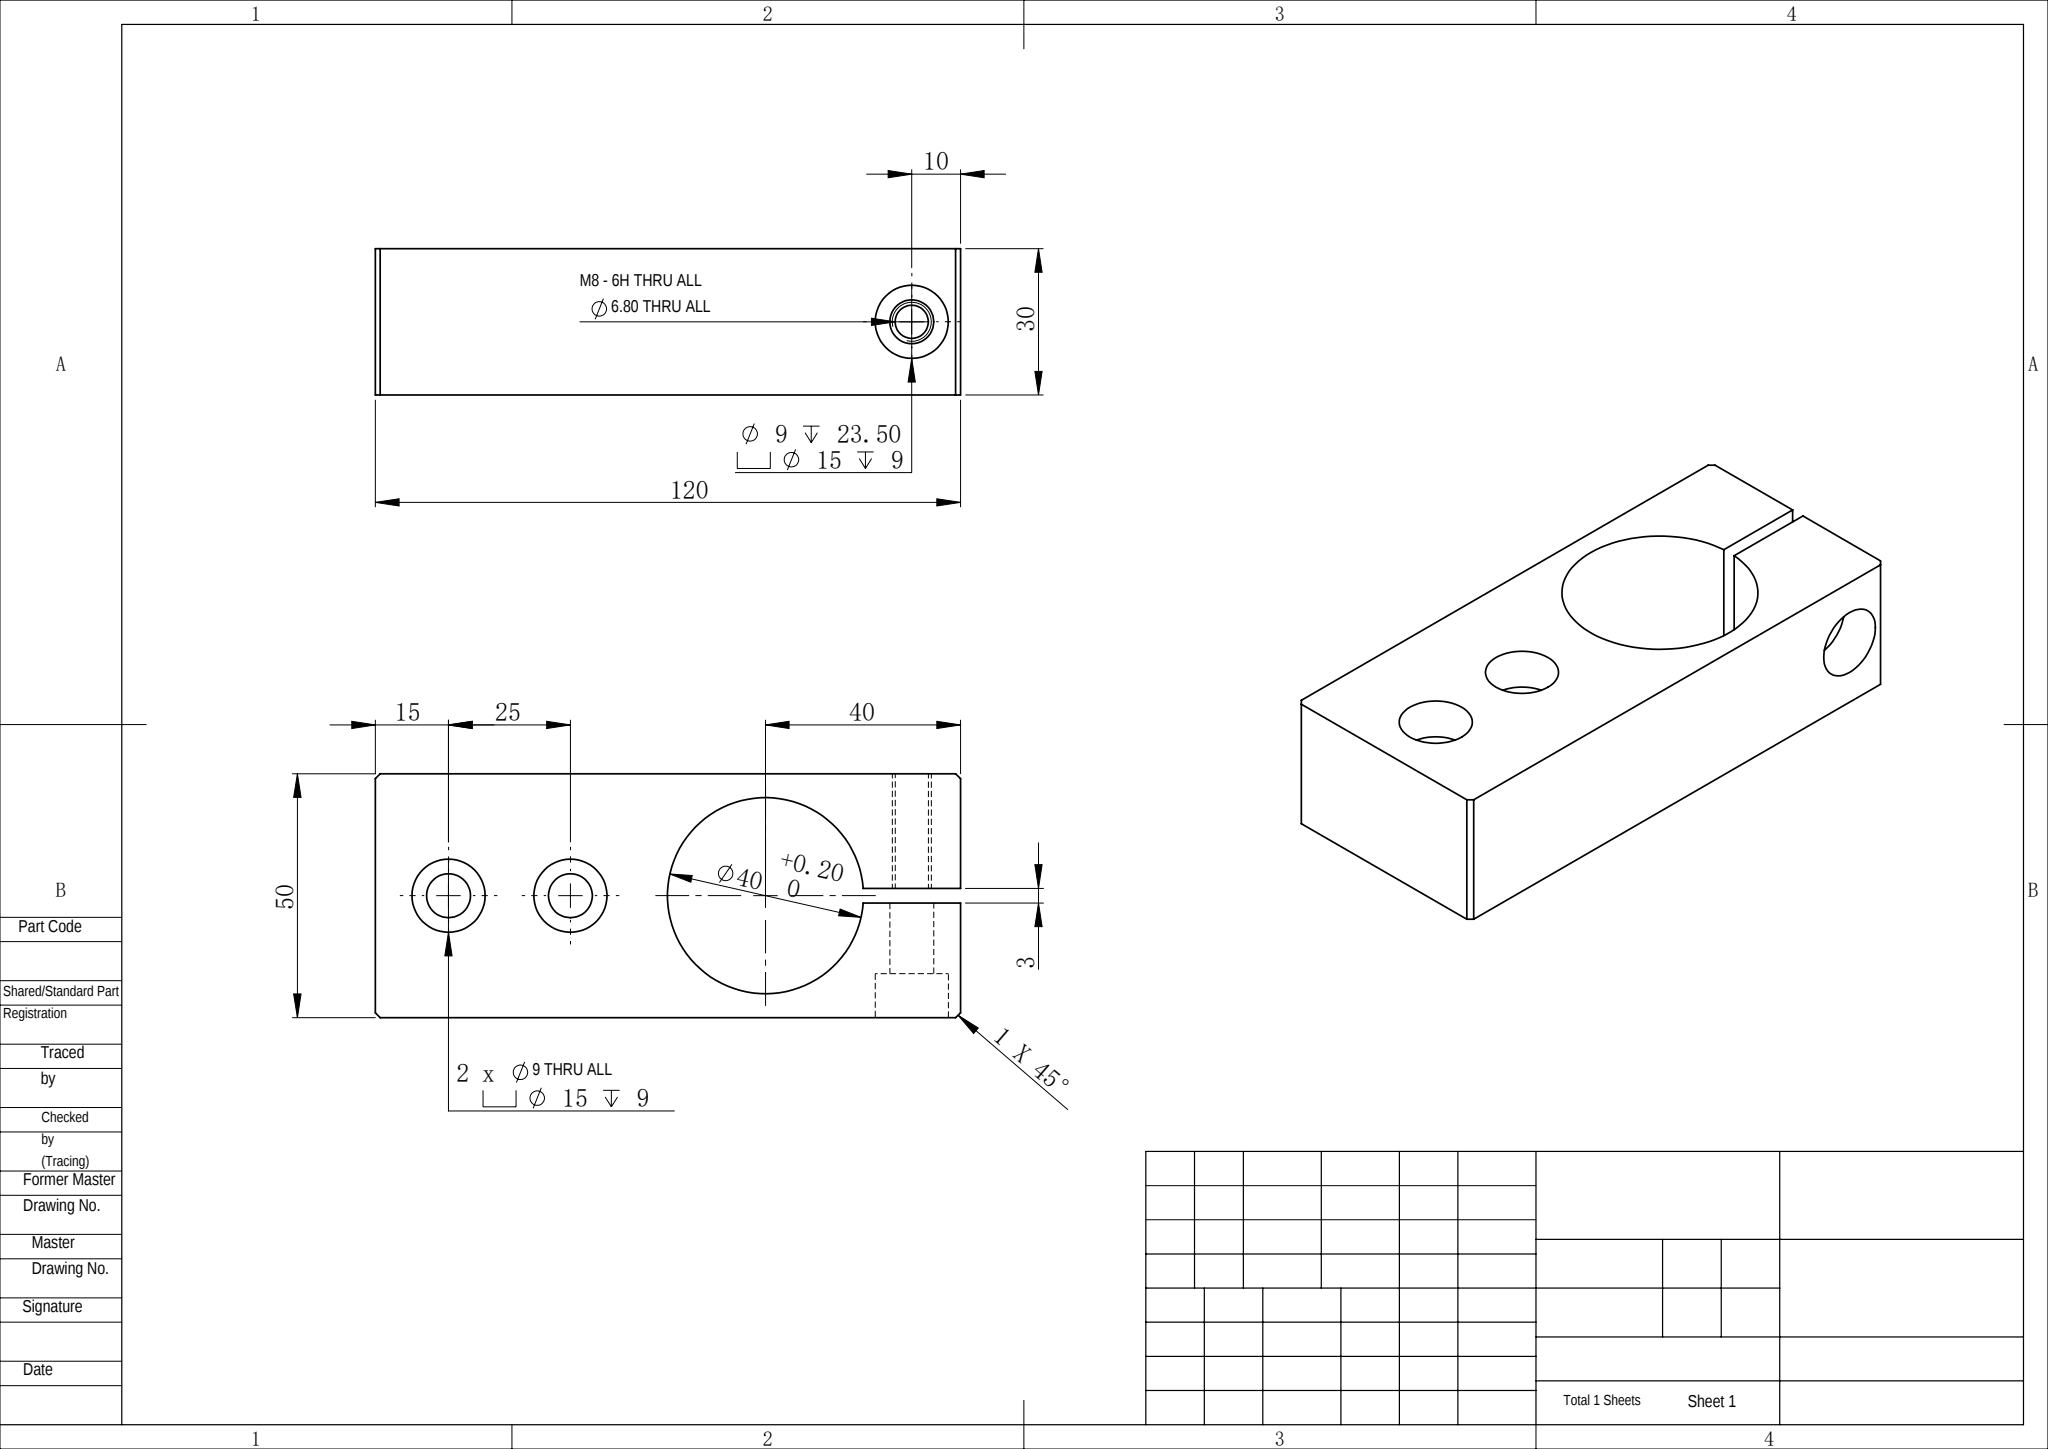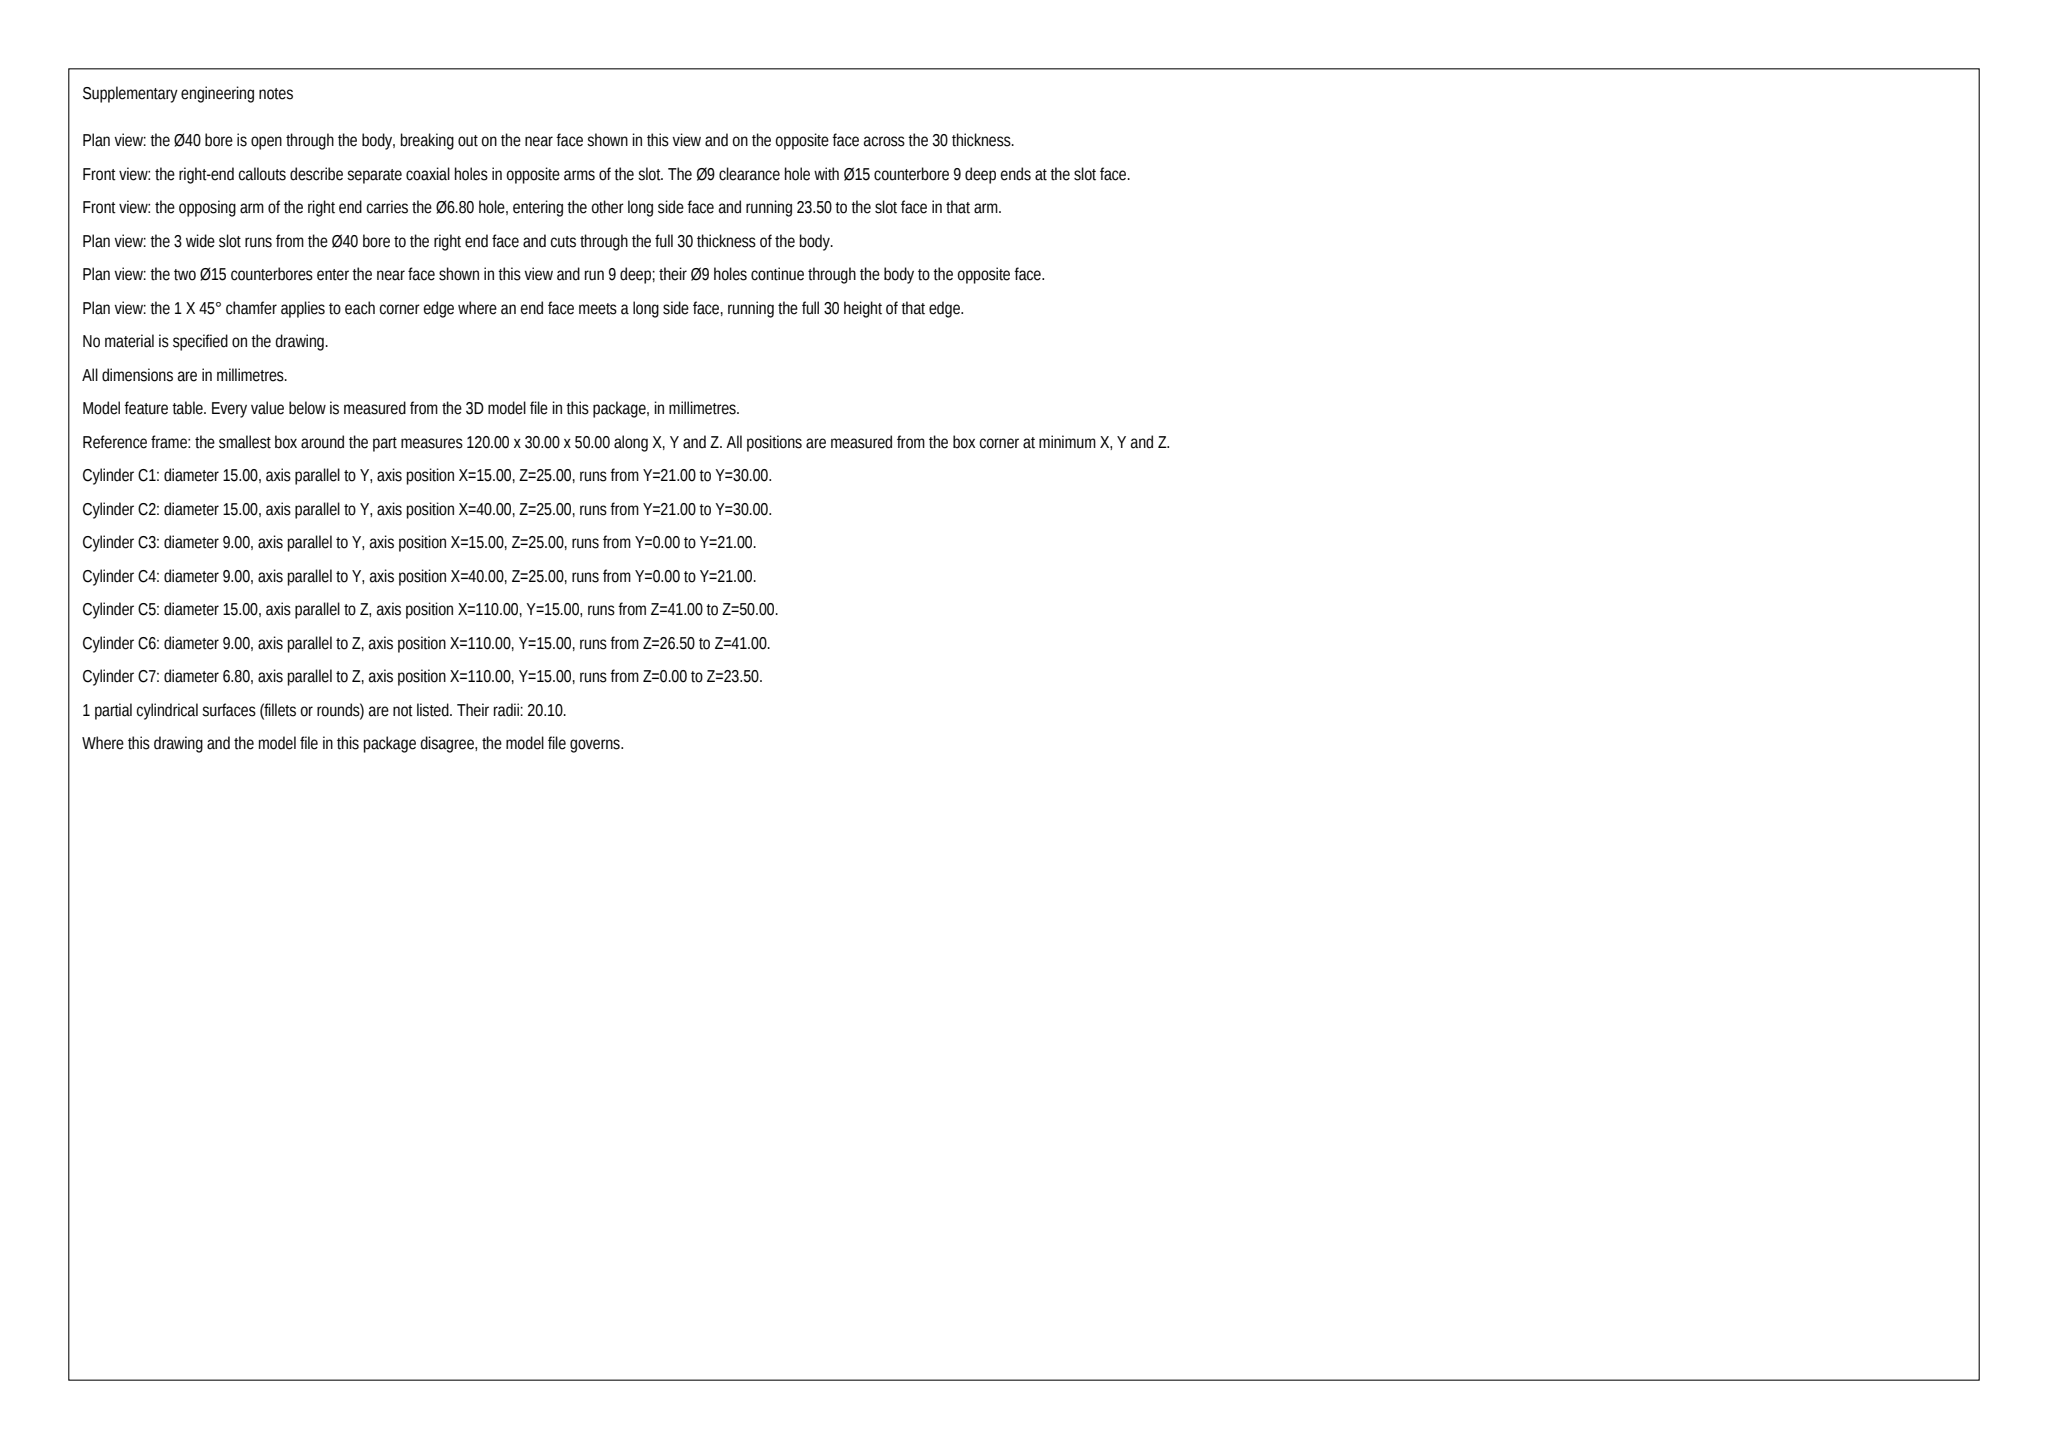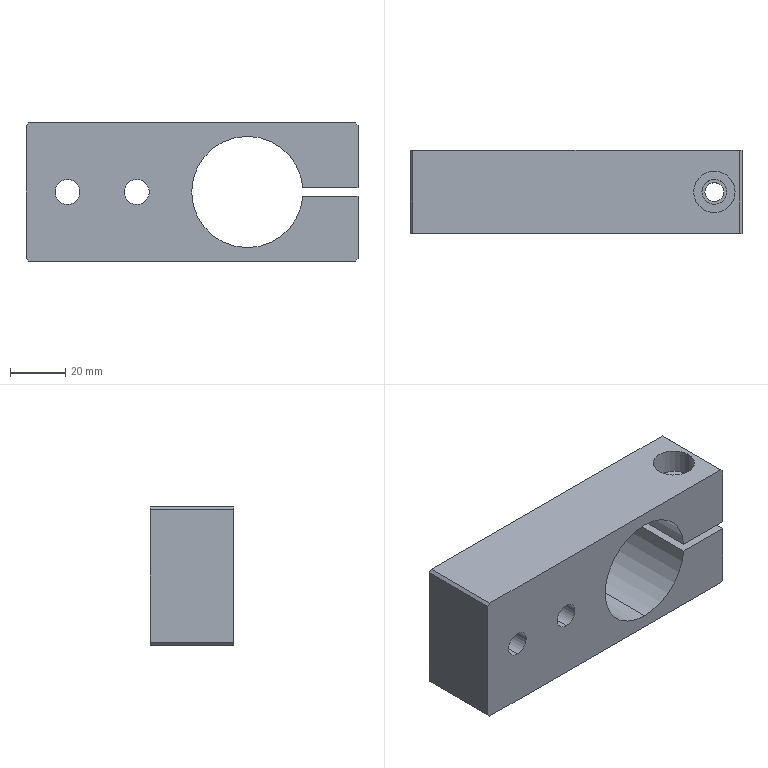Part | SolidWorks | mm | 1 solid | 33 faces | box 120 x 30 x 50 mm | volume 130851 mm3 | cylinder 17 | plane 16 | commonest cylinder face diameters 15 x6 9 x6 40.2 x3 6.8 x2